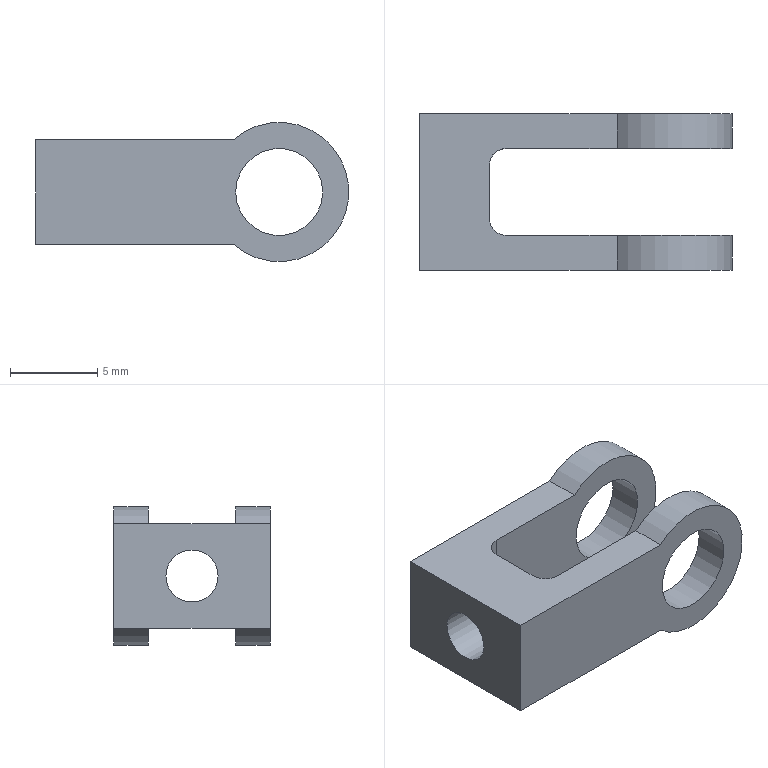Component | NX | LINK_4_BLOCK | 1 solid | 16 faces | volume 467 mm3 | plane 9 | cylinder 7 | commonest cylinder face diameters 8 x2 5 x2 2 x2 3 x1